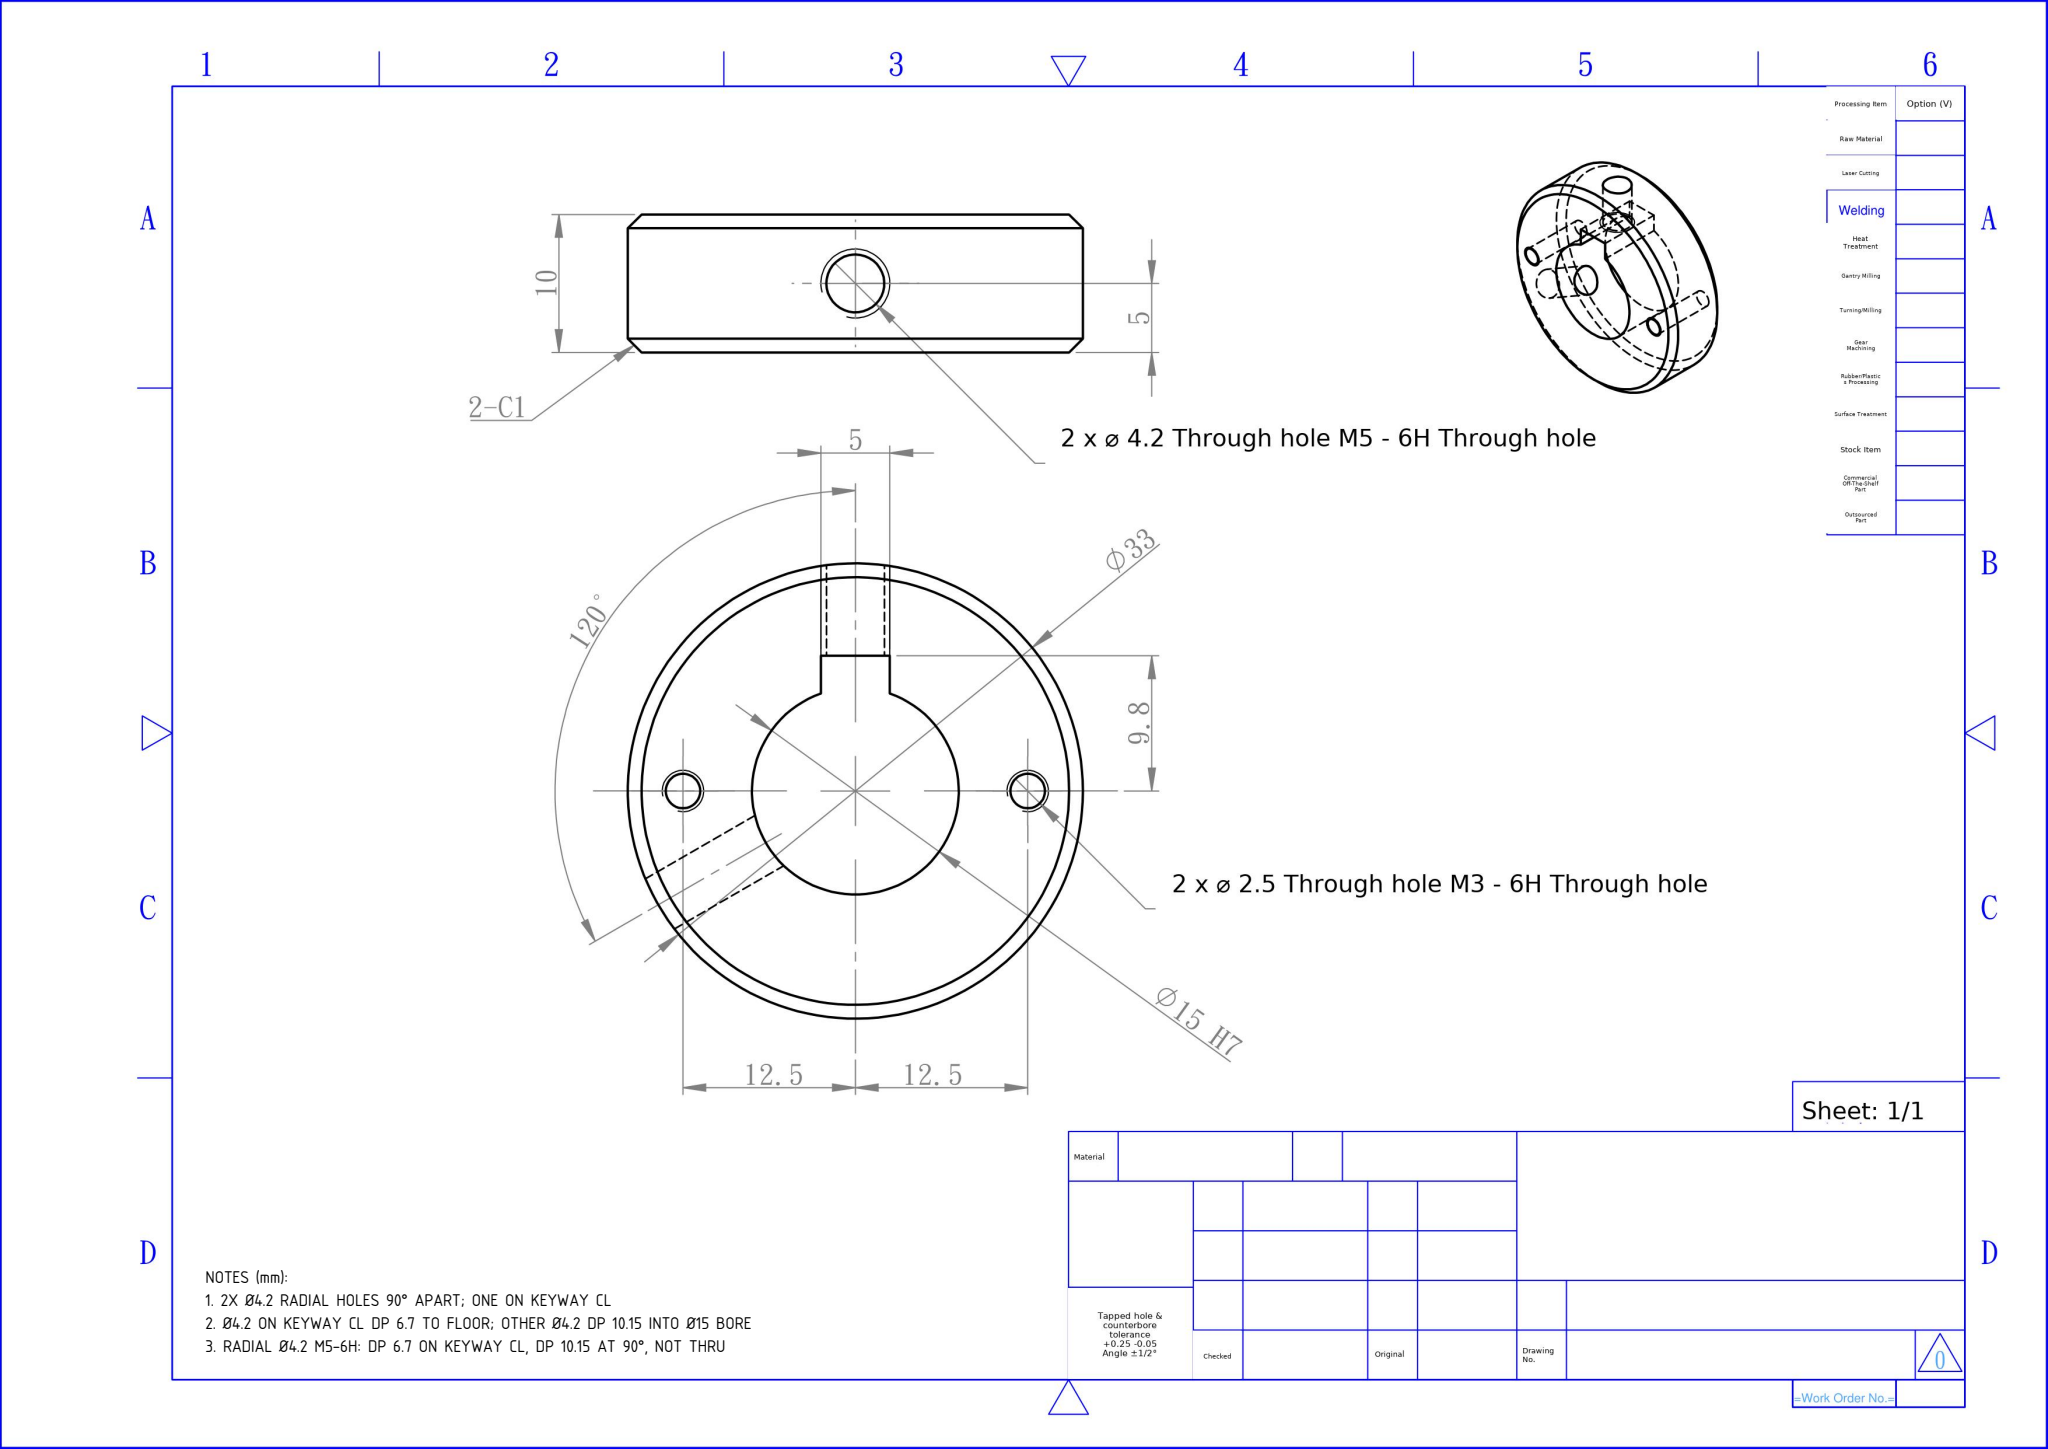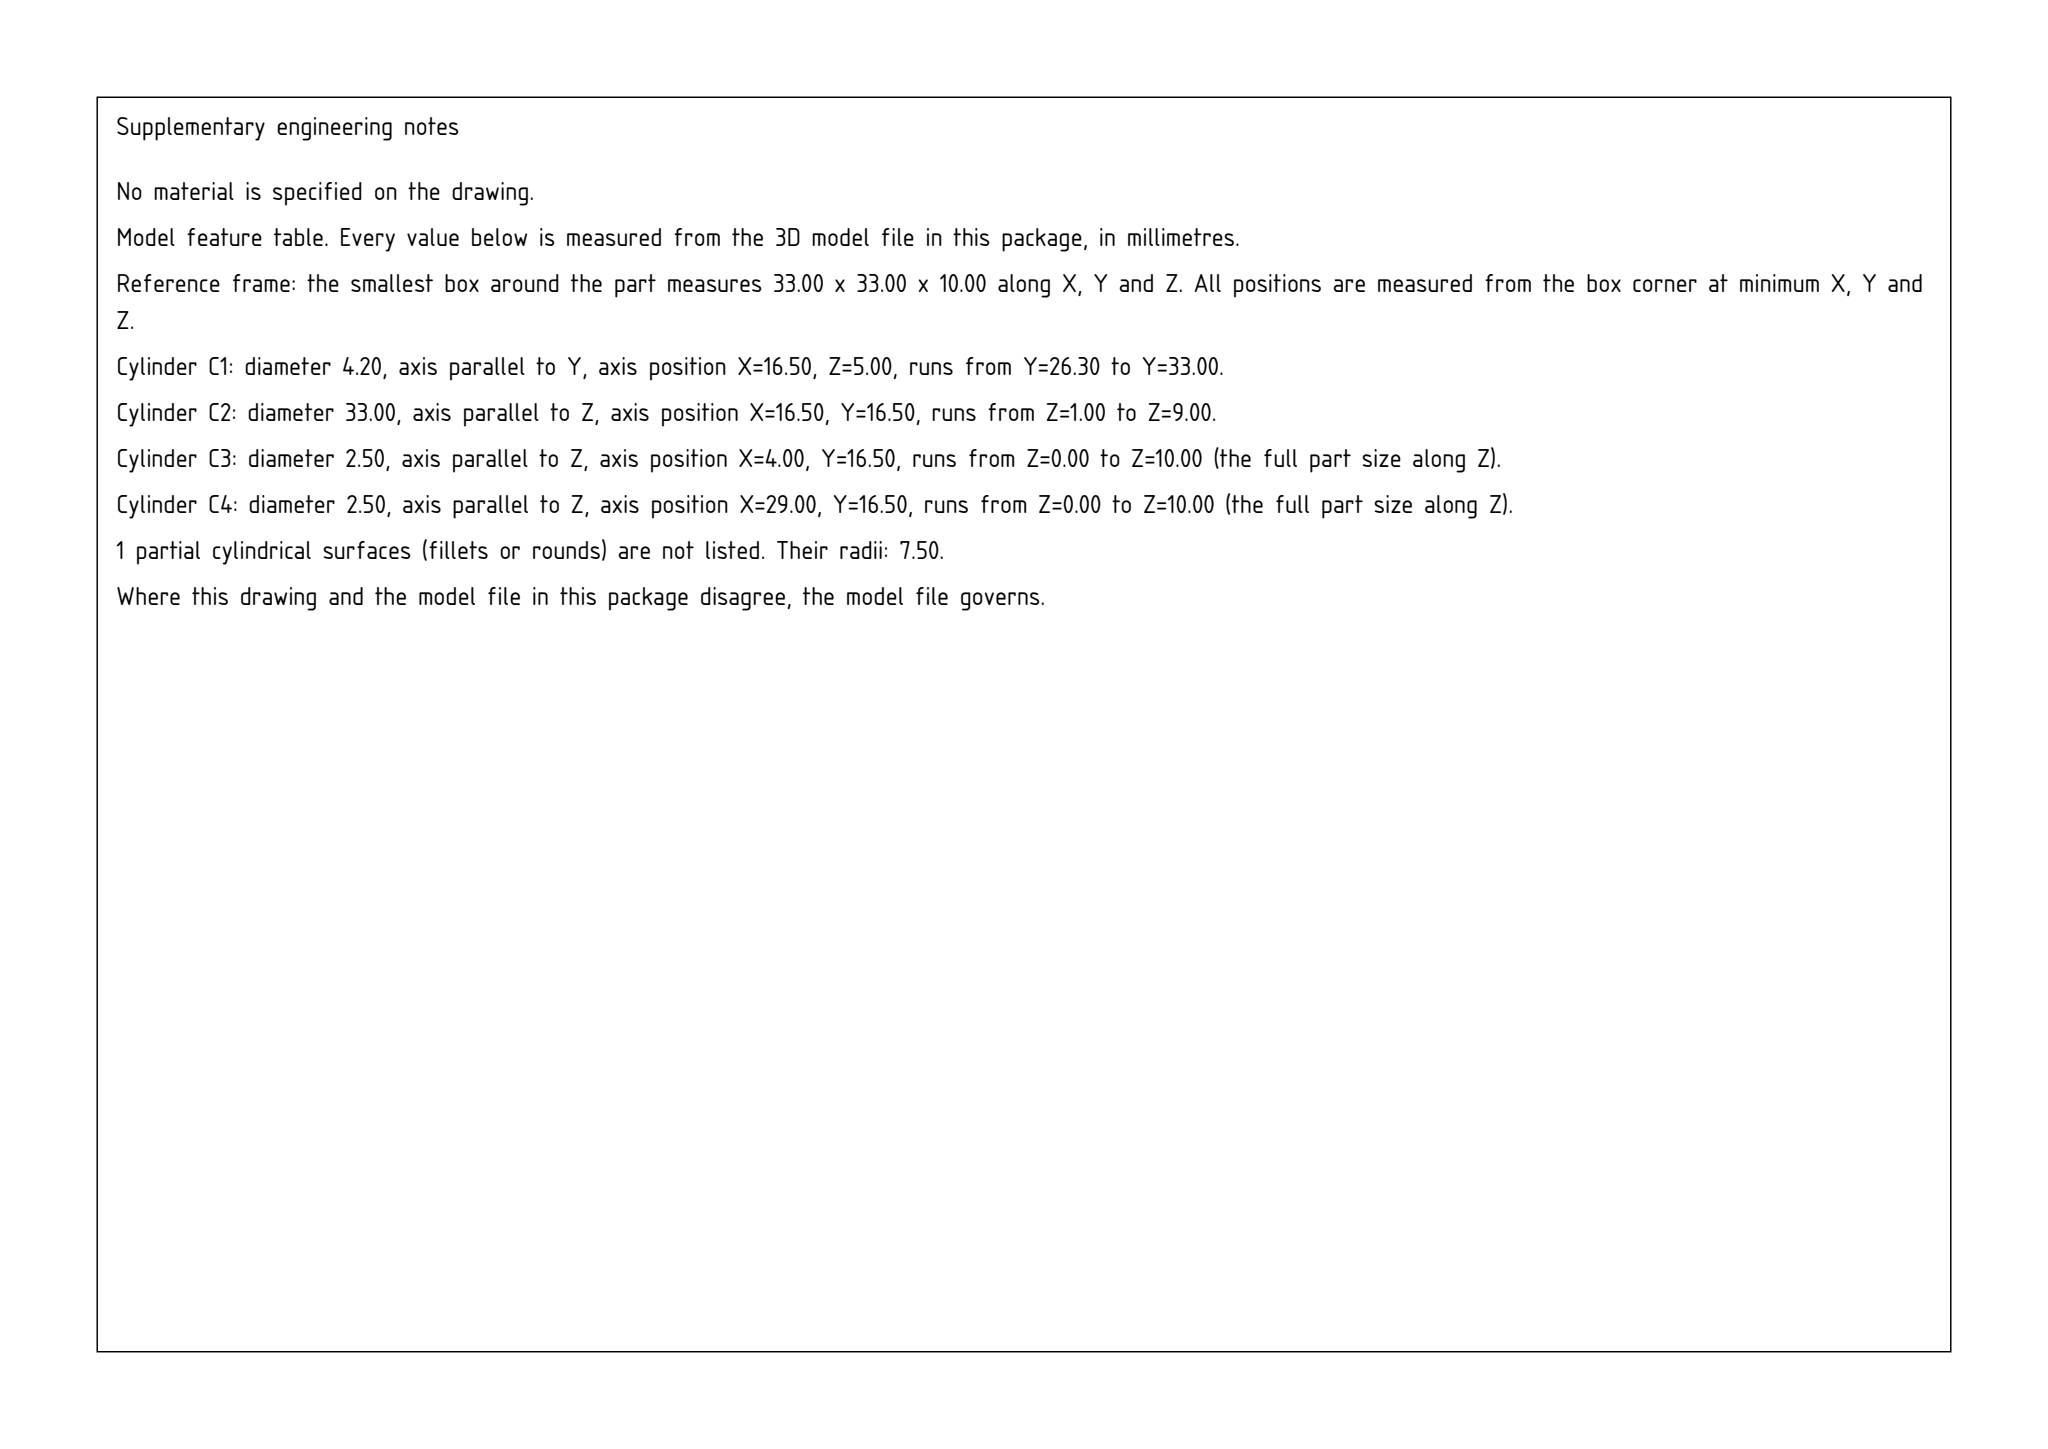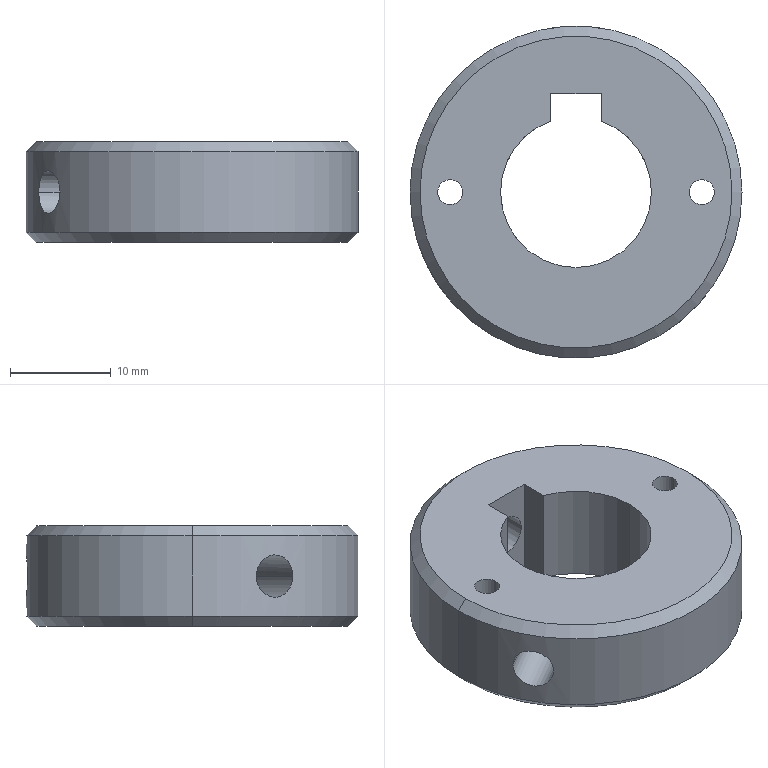Part | SolidWorks | mm | 1 solid | 22 faces | box 33 x 33 x 10 mm | volume 6246 mm3 | cylinder 13 | plane 5 | cone 4 | commonest cylinder face diameters 4.2 x4 2.5 x4 15 x3 33 x2
Drawing notes:
2X Ø4.2 RADIAL HOLES 90° APART; ONE ON KEYWAY CL | from the solid: Ø4.2 cyls: axis X at (y=16.5,z=5) and axis Y at (x=16.5,z=5) - axes perpendicular, Y-axis hole on keyway CL (keyway x=14..19 ctr 16.5)
Ø4.2 ON KEYWAY CL DP 6.7 TO FLOOR; OTHER Ø4.2 DP 10.15 INTO Ø15 BORE | from the solid: Ø4.2 axis Y length 6.7 ends at keyway floor plane y=26.3; Ø4.2 axis X length 10.15 breaks into Ø15 bore at (16.5,16.5)
RADIAL Ø4.2 M5-6H: DP 6.7 ON KEYWAY CL, DP 10.15 AT 90°, NOT THRU | from the solid: cylinders [4.2,'y',[16.5,null,5.0],6.7] and [4.2,'x',[null,16.5,5.0],10.15]
build123d program:
from build123d import *

# Parameters (mm, degrees)
SKETCH1_R               = 16.5
BOSS_EXTRUDE1_DEPTH     = 5
M3_TAPPED_HOLE1_D       = 2.5
SKETCH5_W               = 2.1
SKETCH5_H               = 16.5
CHAMFER1_SIZE           = 1
CIRCULAR_PATTERN1_COUNT = 2
CIRCULAR_PATTERN1_ANGLE = 120


with BuildPart() as part:
    # Sketch1 → Boss-Extrude1 (new, symmetric)
    with BuildSketch(Plane.XY):
        Circle(SKETCH1_R)
        with BuildLine():
            Line((-2.5, 9.8), (2.5, 9.8))
            Line((2.5, 9.8), (2.5, 7.071))
            ThreePointArc((2.5, 7.071), (0, -7.5), (-2.5, 7.071))
            Line((-2.5, 7.071), (-2.5, 9.8))
        make_face(mode=Mode.SUBTRACT)
    extrude(amount=BOSS_EXTRUDE1_DEPTH, both=True)

    # M3 Tapped Hole1 (through all)
    with Locations(Plane.XY.offset(5)):
        with Locations((-12.5, 0), (12.5, 0)):
            Hole(M3_TAPPED_HOLE1_D / 2)

    # Sketch5 → M5 Tapped Hole1 (revolve, cut)
    with BuildSketch(Plane(origin=(0, 0, 0), x_dir=(0, 0, -1), z_dir=(1, 0, 0))):
        with Locations((1.05, 8.25)):
            Rectangle(SKETCH5_W, SKETCH5_H)
    m5_tapped_hole1 = revolve(axis=Axis((0, -6.35, 0), (0, 1, 0)), mode=Mode.SUBTRACT)

    # Chamfer1
    chamfer1_edges = [part.edges().sort_by_distance(p)[0] for p in [
        (-16.5, 0, -5),
        (-16.5, 0, 5),
    ]]
    chamfer(chamfer1_edges, length=CHAMFER1_SIZE)

    # Circular Pattern1: M5 Tapped Hole1 ×2 about axis
    circular_pattern1_axis = Axis((0, 0, 5), (0, 0, 1))
    for i in range(1, CIRCULAR_PATTERN1_COUNT):
        add(m5_tapped_hole1.rotate(circular_pattern1_axis, i * CIRCULAR_PATTERN1_ANGLE / (CIRCULAR_PATTERN1_COUNT - 1)), mode=Mode.SUBTRACT)


solid = part.part